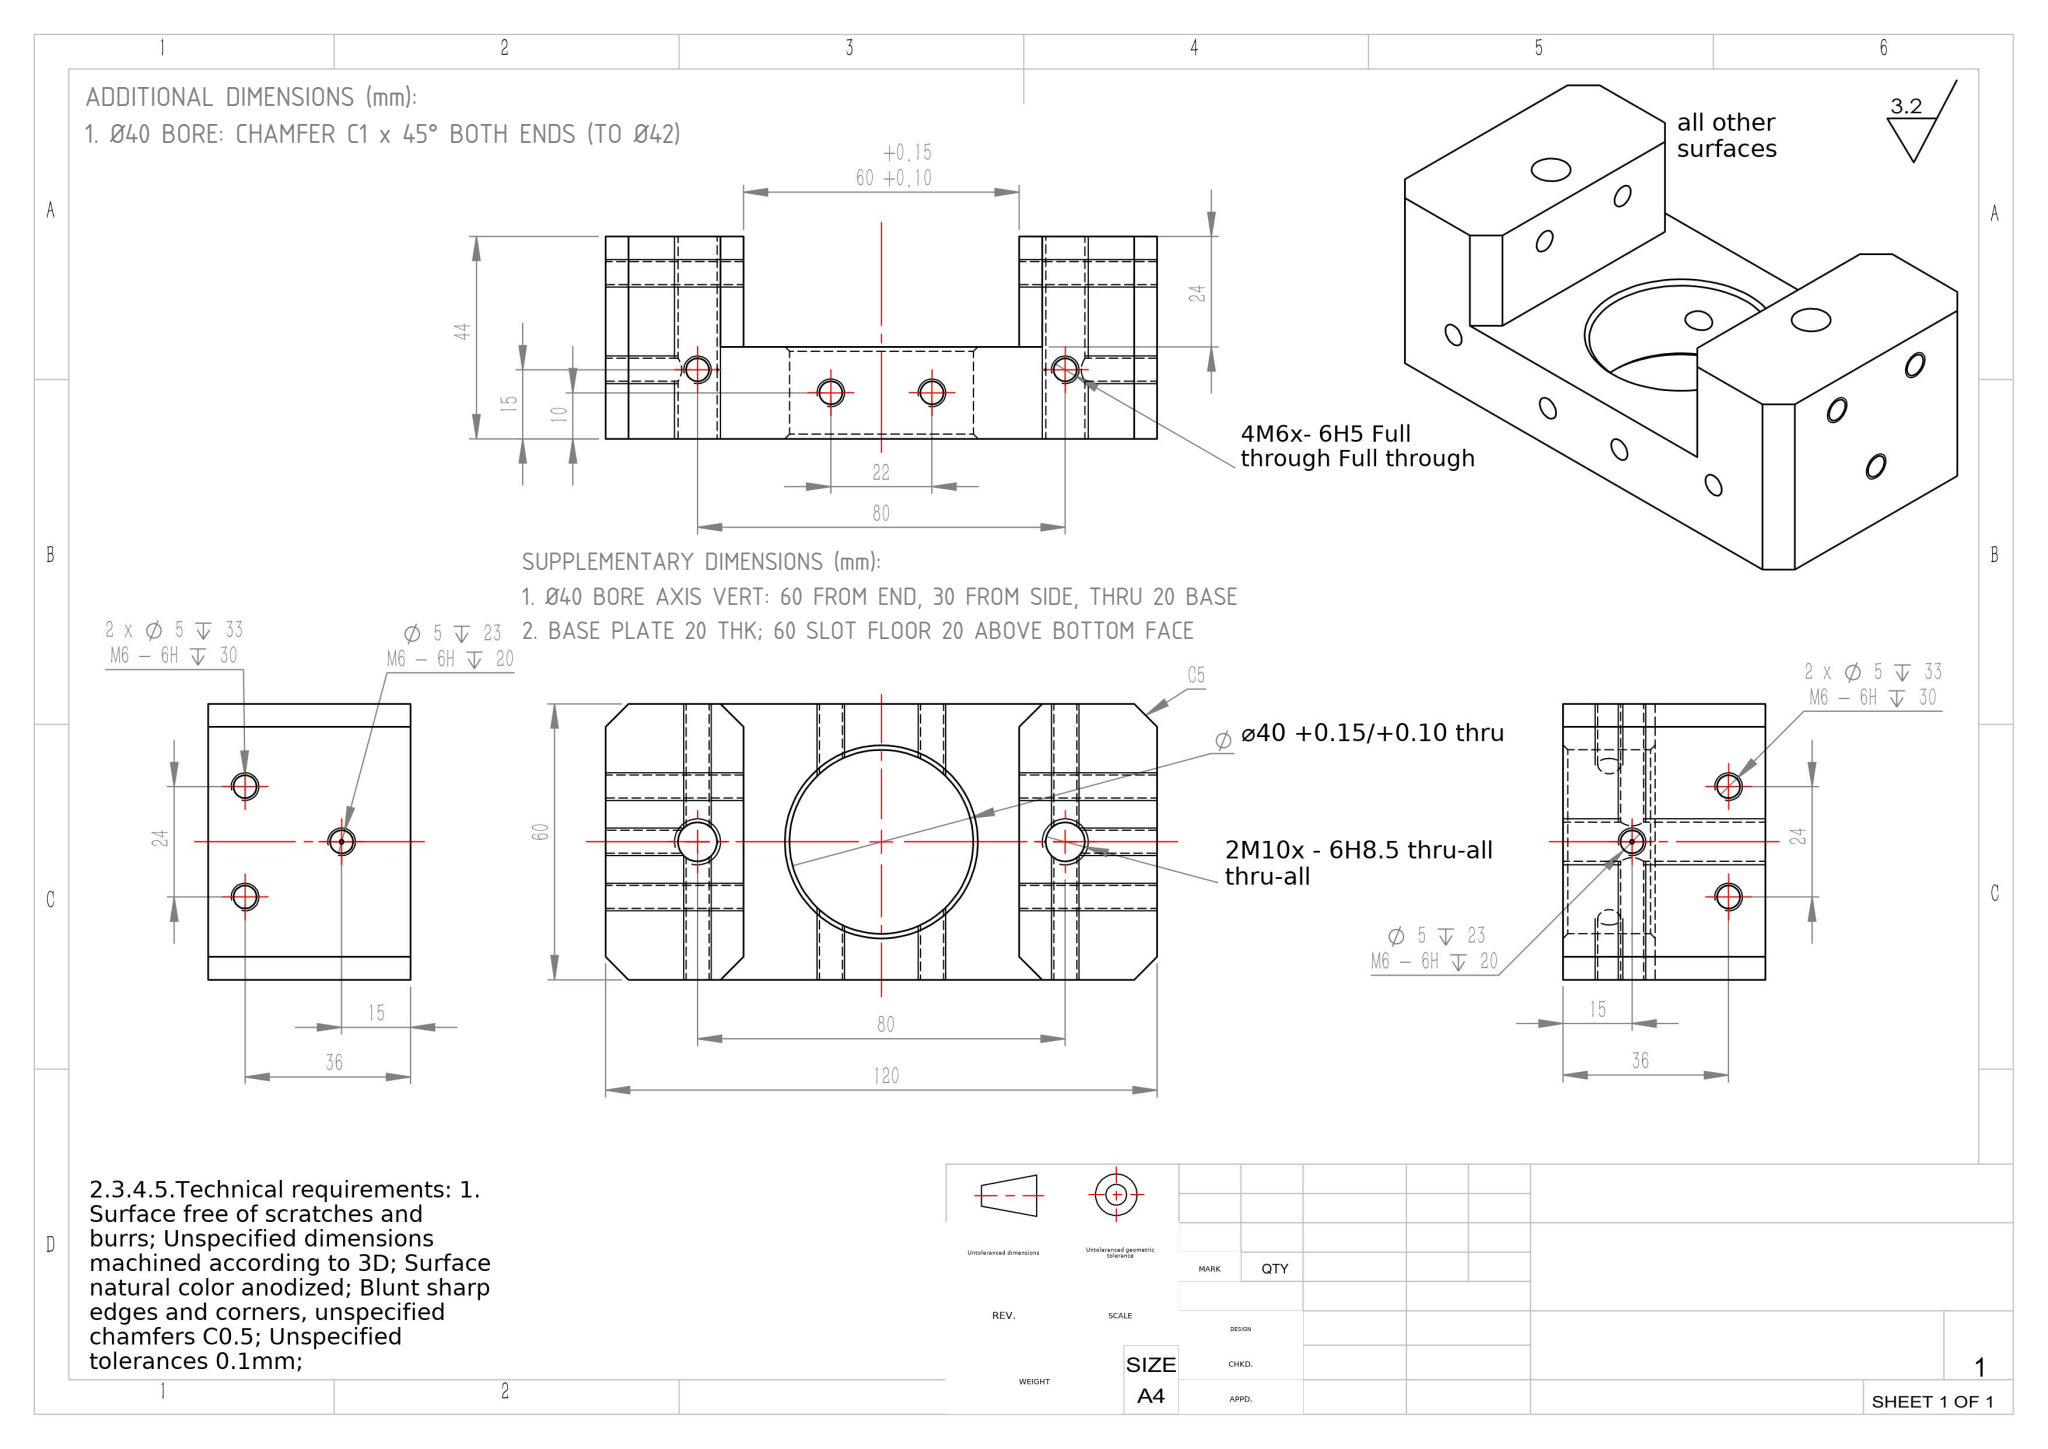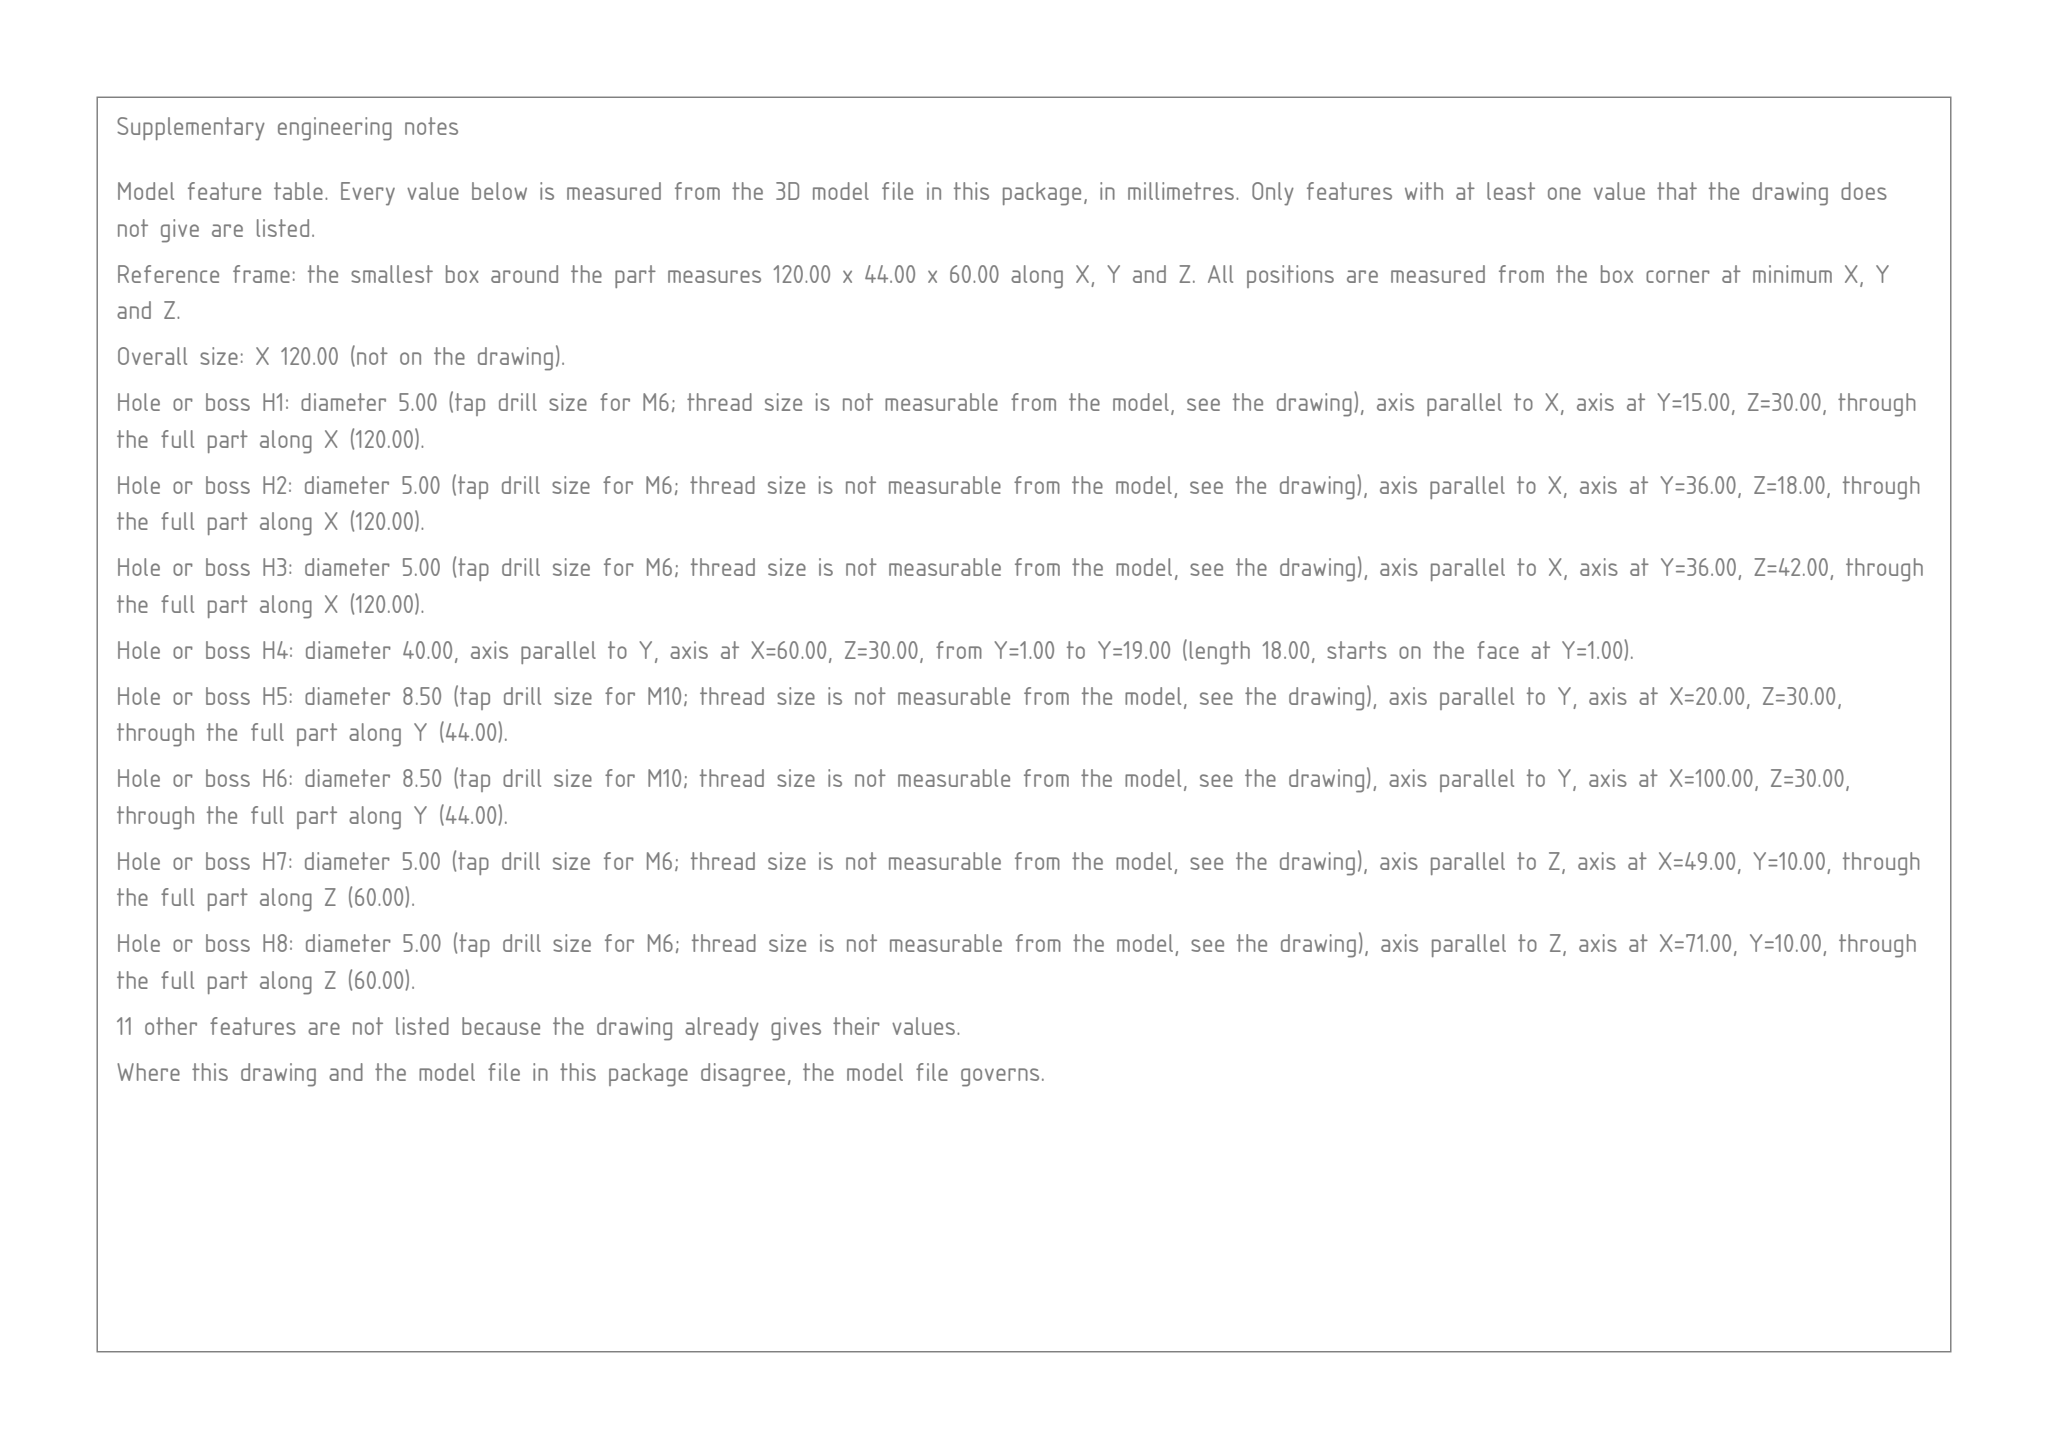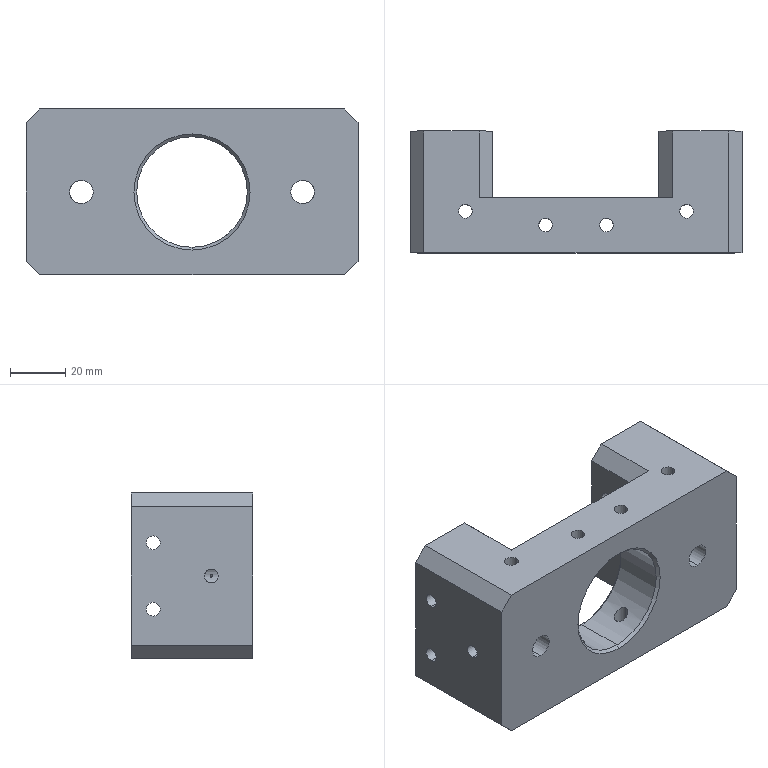Part | SolidWorks | mm | 1 solid | 60 faces | box 120 x 44 x 60 mm | volume 190676 mm3 | cylinder 34 | plane 18 | cone 8 | commonest cylinder face diameters 5 x28 8.5 x4 40 x2
build123d program:
from build123d import *

# Parameters (mm, degrees)
SKETCH1_W             = 120
SKETCH1_H             = 60
BOSS_EXTRUDE1_DEPTH   = 44
SKETCH2_R             = 20
CUT_EXTRUDE1_DEPTH    = 81.225
SKETCH3_W             = 60
SKETCH3_H             = 60
CUT_EXTRUDE2_DEPTH    = 24
M10_TAPPED_HOLE1_D    = 8.5
M6_TAPPED_HOLE1_D     = 5
M6_TAPPED_HOLE2_D     = 5
M6_TAPPED_HOLE2_DEPTH = 23
M6_TAPPED_HOLE2_TIP   = 1.502
M6_TAPPED_HOLE3_D     = 5
M6_TAPPED_HOLE3_DEPTH = 23
M6_TAPPED_HOLE3_TIP   = 1.502
CHAMFER1_SIZE         = 5
M6_TAPPED_HOLE4_D     = 5
M6_TAPPED_HOLE4_DEPTH = 33
M6_TAPPED_HOLE4_TIP   = 1.502
M6_TAPPED_HOLE5_D     = 5
M6_TAPPED_HOLE5_DEPTH = 33
M6_TAPPED_HOLE5_TIP   = 1.502
CHAMFER2_SIZE         = 1


with BuildPart() as part:
    # Sketch1 → Boss-Extrude1 (new body)
    with BuildSketch(Plane(origin=(0, 0, 0), x_dir=(1, 0, 0), z_dir=(0, 1, 0))):
        Rectangle(SKETCH1_W, SKETCH1_H)
    extrude(amount=BOSS_EXTRUDE1_DEPTH)

    # Sketch2 → Cut-Extrude1 (cut, through all)
    with BuildSketch(Plane(origin=(0, 44, 0), x_dir=(1, 0, 0), z_dir=(0, 1, 0))):
        with Locations(Location((0, 0, 0), (0, 0, 270))):
            Circle(SKETCH2_R)
    extrude(amount=-CUT_EXTRUDE1_DEPTH, mode=Mode.SUBTRACT)

    # Sketch3 → Cut-Extrude2 (cut)
    with BuildSketch(Plane(origin=(0, 44, 0), x_dir=(1, 0, 0), z_dir=(0, 1, 0))):
        Rectangle(SKETCH3_W, SKETCH3_H)
    extrude(amount=-CUT_EXTRUDE2_DEPTH, mode=Mode.SUBTRACT)

    # M10 Tapped Hole1 (through all)
    with Locations(Plane(origin=(0, 0, 0), x_dir=(-1, 0, 0), z_dir=(0, -1, 0))):
        with Locations((-40, 0), (40, 0)):
            Hole(M10_TAPPED_HOLE1_D / 2)

    # M6 Tapped Hole1 (through all)
    with Locations(Plane(origin=(0, 0, -30), x_dir=(-1, 0, 0), z_dir=(0, 0, -1))):
        with Locations((-40, 15), (40, 15), (-11, 10), (11, 10)):
            Hole(M6_TAPPED_HOLE1_D / 2)

    # M6 Tapped Hole2
    with Locations(Plane(origin=(60, 0, 0), x_dir=(0, 0, -1), z_dir=(1, 0, 0))):
        with Locations((0, 15)):
            Hole(M6_TAPPED_HOLE2_D / 2, depth=M6_TAPPED_HOLE2_DEPTH)
            with Locations((0, 0, -(M6_TAPPED_HOLE2_DEPTH + M6_TAPPED_HOLE2_TIP / 2))):  # 118° drill point
                Cone(0, M6_TAPPED_HOLE2_D / 2, M6_TAPPED_HOLE2_TIP, mode=Mode.SUBTRACT)

    # M6 Tapped Hole3
    with Locations(Plane.ZY.offset(60)):
        with Locations((0, 15)):
            Hole(M6_TAPPED_HOLE3_D / 2, depth=M6_TAPPED_HOLE3_DEPTH)
            with Locations((0, 0, -(M6_TAPPED_HOLE3_DEPTH + M6_TAPPED_HOLE3_TIP / 2))):  # 118° drill point
                Cone(0, M6_TAPPED_HOLE3_D / 2, M6_TAPPED_HOLE3_TIP, mode=Mode.SUBTRACT)

    # Chamfer1
    chamfer1_edges = [part.edges().sort_by_distance(p)[0] for p in [
        (30, 32, -30),
        (30, 32, 30),
        (-30, 32, 30),
        (-30, 32, -30),
        (60, 22, 30),
        (-60, 22, 30),
        (-60, 22, -30),
        (60, 22, -30),
    ]]
    chamfer(chamfer1_edges, length=CHAMFER1_SIZE)

    # M6 Tapped Hole4
    with Locations(Plane.ZY.offset(60)):
        with Locations((-12, 36), (12, 36)):
            Hole(M6_TAPPED_HOLE4_D / 2, depth=M6_TAPPED_HOLE4_DEPTH)
            with Locations((0, 0, -(M6_TAPPED_HOLE4_DEPTH + M6_TAPPED_HOLE4_TIP / 2))):  # 118° drill point
                Cone(0, M6_TAPPED_HOLE4_D / 2, M6_TAPPED_HOLE4_TIP, mode=Mode.SUBTRACT)

    # M6 Tapped Hole5
    with Locations(Plane(origin=(60, 0, 0), x_dir=(0, 0, -1), z_dir=(1, 0, 0))):
        with Locations((-12, 36), (12, 36)):
            Hole(M6_TAPPED_HOLE5_D / 2, depth=M6_TAPPED_HOLE5_DEPTH)
            with Locations((0, 0, -(M6_TAPPED_HOLE5_DEPTH + M6_TAPPED_HOLE5_TIP / 2))):  # 118° drill point
                Cone(0, M6_TAPPED_HOLE5_D / 2, M6_TAPPED_HOLE5_TIP, mode=Mode.SUBTRACT)

    # Chamfer2
    chamfer2_edges = [part.edges().sort_by_distance(p)[0] for p in [
        (0, 0, -20),
        (0, 20, -20),
    ]]
    chamfer(chamfer2_edges, length=CHAMFER2_SIZE)


solid = part.part